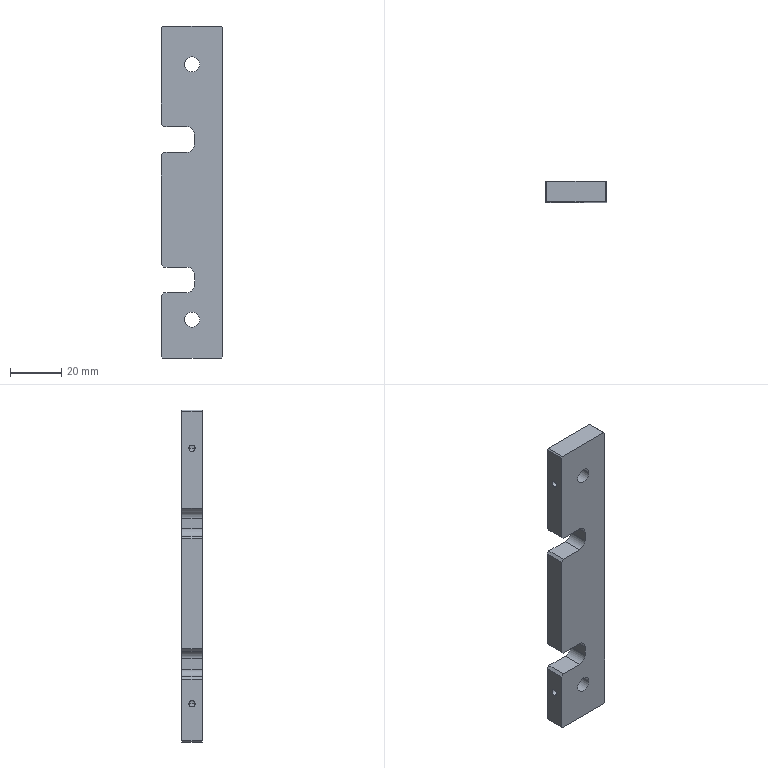Component | SolidWorks | LH-CGJ-01-054-1 | 1 solid | 34 faces | box 24 x 8 x 130 mm | volume 22380 mm3 | plane 22 | cylinder 12 | commonest cylinder face diameters 6 x8 2.5 x4 | material A6061
build123d program:
from build123d import *

# Parameters (mm, degrees)
SKETCH1_W             = 130
SKETCH1_H             = 24
BOSS_EXTRUDE1_DEPTH   = 8
M6_TAPPED_HOLE1_D     = 6
M6_TAPPED_HOLE1_DEPTH = 15
M6_TAPPED_HOLE1_TIP   = 1.803
CHAMFER1_SIZE         = 0.5
M3_TAPPED_HOLE1_D     = 2.5
M3_TAPPED_HOLE1_DEPTH = 12
M3_TAPPED_HOLE1_TIP   = 0.7511
CUT_EXTRUDE1_DEPTH    = 10
LPATTERN1_COUNT       = 2
LPATTERN1_PITCH       = 55
CHAMFER2_SIZE         = 1


with BuildPart() as part:
    # Sketch1 → Boss-Extrude1 (new body)
    with BuildSketch(Plane(origin=(0, 0, 0), x_dir=(1, 0, 0), z_dir=(0, 1, 0))):
        with Locations((65, 12)):
            Rectangle(SKETCH1_W, SKETCH1_H)
    extrude(amount=BOSS_EXTRUDE1_DEPTH)

    # M6 Tapped Hole1
    with Locations(Plane(origin=(0, 8, 0), x_dir=(1, 0, 0), z_dir=(0, 1, 0))):
        with Locations((15, 12), (115, 12)):
            Hole(M6_TAPPED_HOLE1_D / 2, depth=M6_TAPPED_HOLE1_DEPTH)
            with Locations((0, 0, -(M6_TAPPED_HOLE1_DEPTH + M6_TAPPED_HOLE1_TIP / 2))):  # 118° drill point
                Cone(0, M6_TAPPED_HOLE1_D / 2, M6_TAPPED_HOLE1_TIP, mode=Mode.SUBTRACT)

    # Chamfer1
    chamfer1_edges = [part.edges().sort_by_distance(p)[0] for p in [
        (0, 4, -24),
        (130, 4, -24),
        (130, 4, 0),
        (0, 4, 0),
    ]]
    chamfer(chamfer1_edges, length=CHAMFER1_SIZE)

    # M3 Tapped Hole1
    with Locations(Plane(origin=(0, 0, -24), x_dir=(-1, 0, 0), z_dir=(0, 0, -1))):
        with Locations((-115, 4), (-15, 4)):
            Hole(M3_TAPPED_HOLE1_D / 2, depth=M3_TAPPED_HOLE1_DEPTH)
            with Locations((0, 0, -(M3_TAPPED_HOLE1_DEPTH + M3_TAPPED_HOLE1_TIP / 2))):  # 118° drill point
                Cone(0, M3_TAPPED_HOLE1_D / 2, M3_TAPPED_HOLE1_TIP, mode=Mode.SUBTRACT)

    # Sketch6 → Cut-Extrude1 (cut)
    with BuildSketch(Plane(origin=(0, 8, 0), x_dir=(1, 0, 0), z_dir=(0, 1, 0))):
        with BuildLine():
            Line((94.452, 24), (104.452, 24))
            Line((104.452, 24), (104.452, 14))
            ThreePointArc((104.452, 14), (103.573, 11.879), (101.452, 11))
            Line((101.452, 11), (97.452, 11))
            ThreePointArc((97.452, 11), (95.33, 11.879), (94.452, 14))
            Line((94.452, 14), (94.452, 24))
        make_face()
    cut_extrude1 = extrude(amount=-CUT_EXTRUDE1_DEPTH, mode=Mode.SUBTRACT)

    # LPattern1: Cut-Extrude1 ×2
    with Locations(*[(-i * LPATTERN1_PITCH, 0, 0) for i in range(1, LPATTERN1_COUNT)]):
        add(cut_extrude1, mode=Mode.SUBTRACT)

    # Chamfer2
    chamfer2_edges = [part.edges().sort_by_distance(p)[0] for p in [
        (39.452, 4, -24),
        (49.452, 4, -24),
        (94.452, 4, -24),
        (104.452, 4, -24),
    ]]
    chamfer(chamfer2_edges, length=CHAMFER2_SIZE)


solid = part.part

# Placed as in the assembly
solid = solid.moved(Location((-24.003, -16.285, 130.05), (0, 90, 0)))